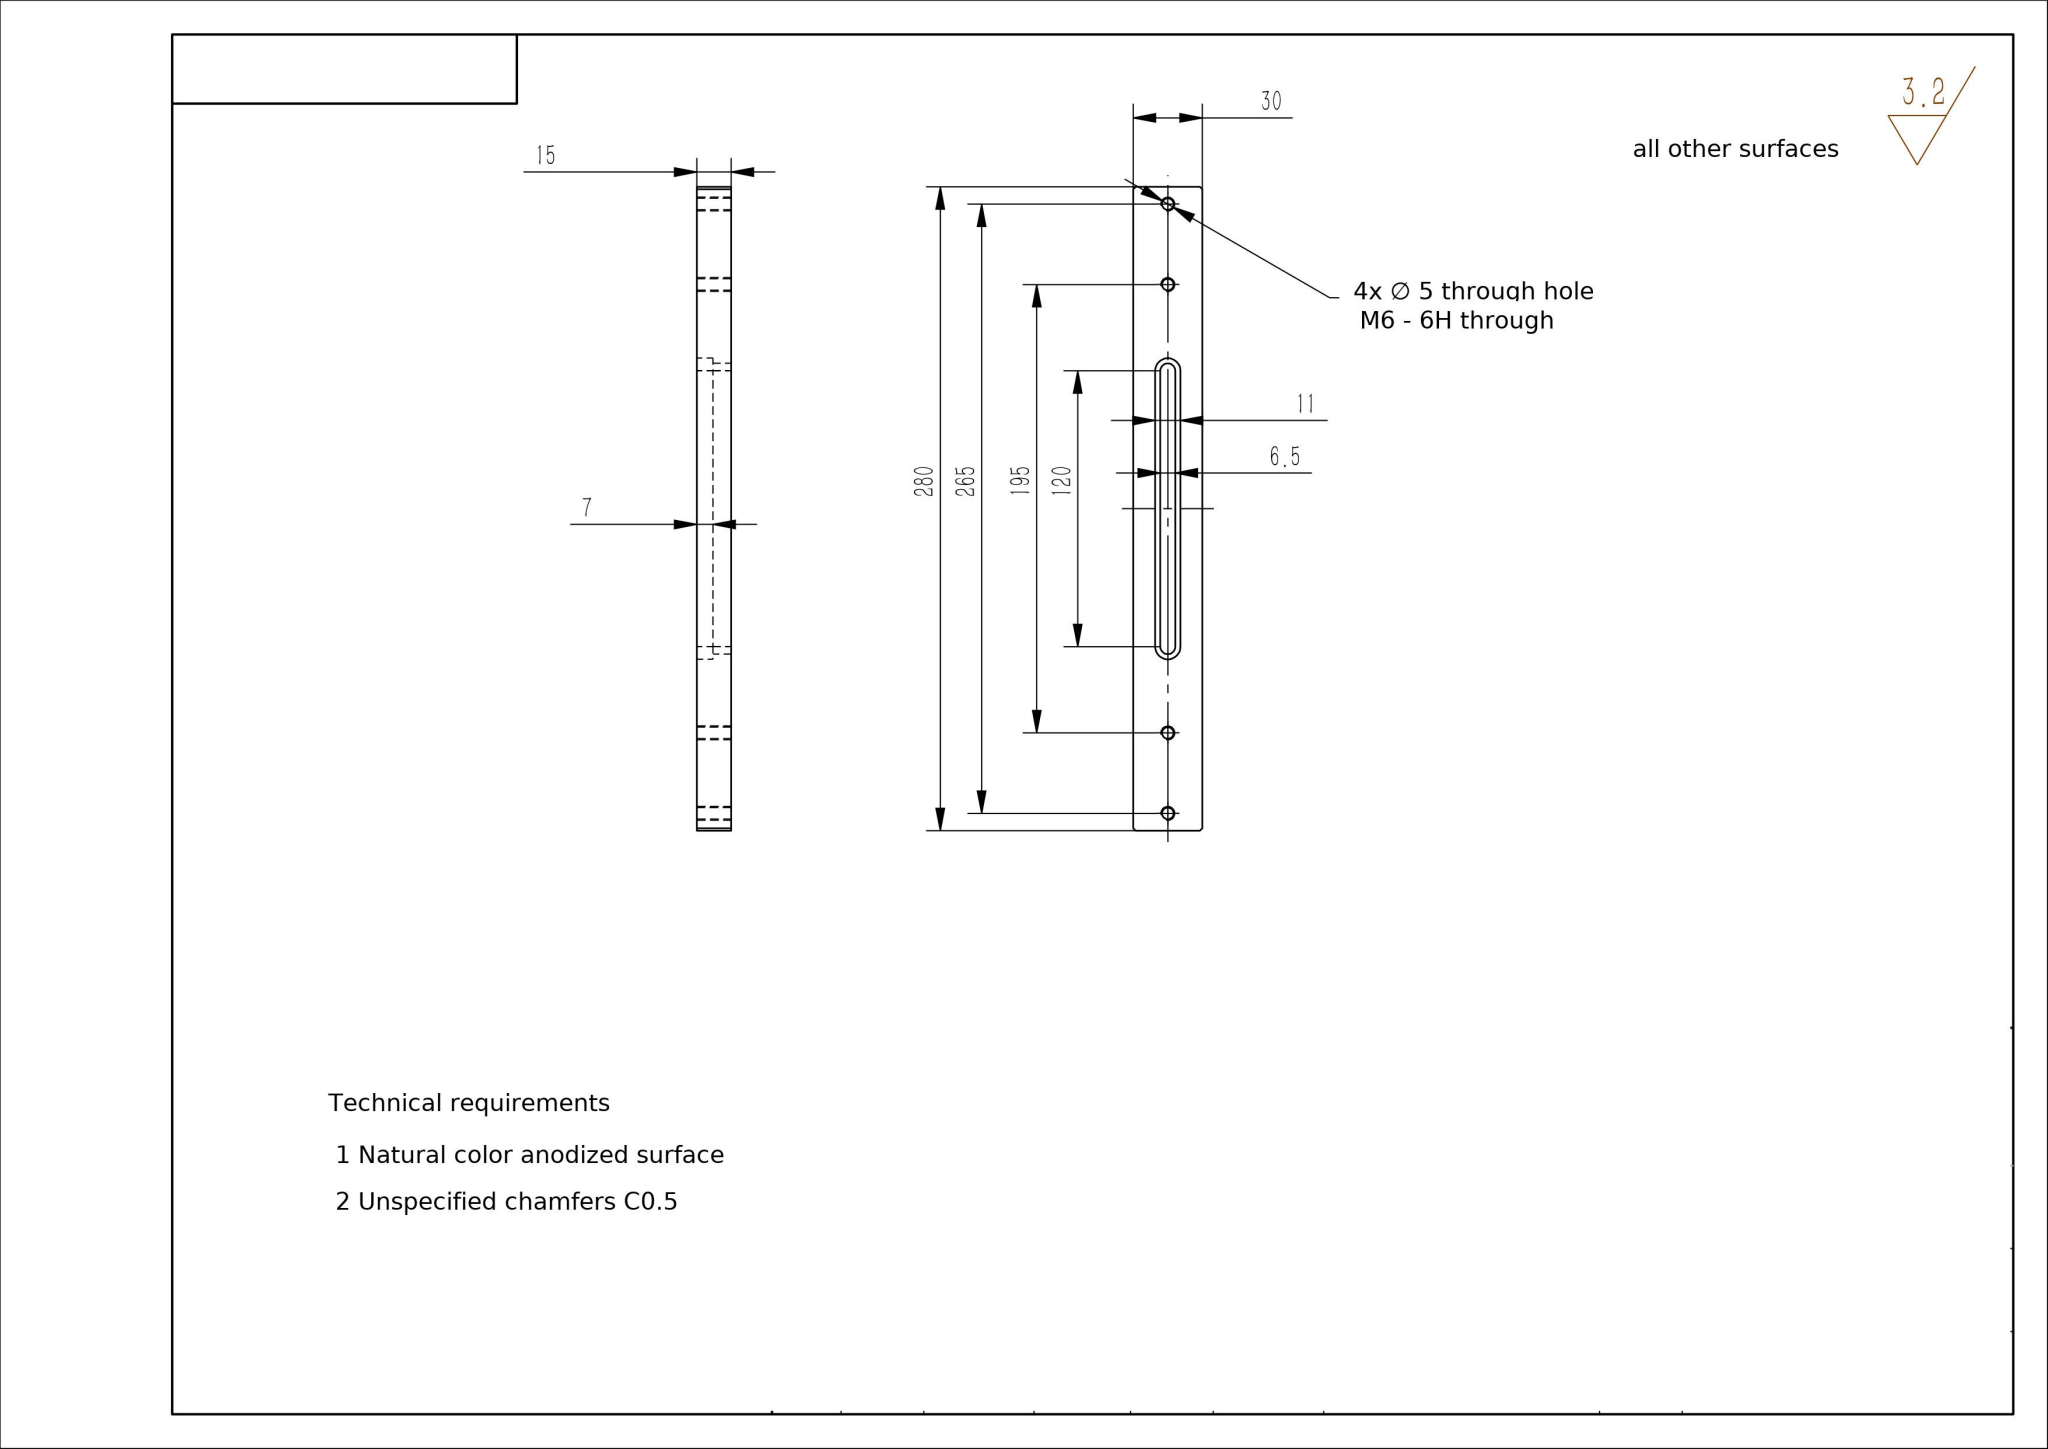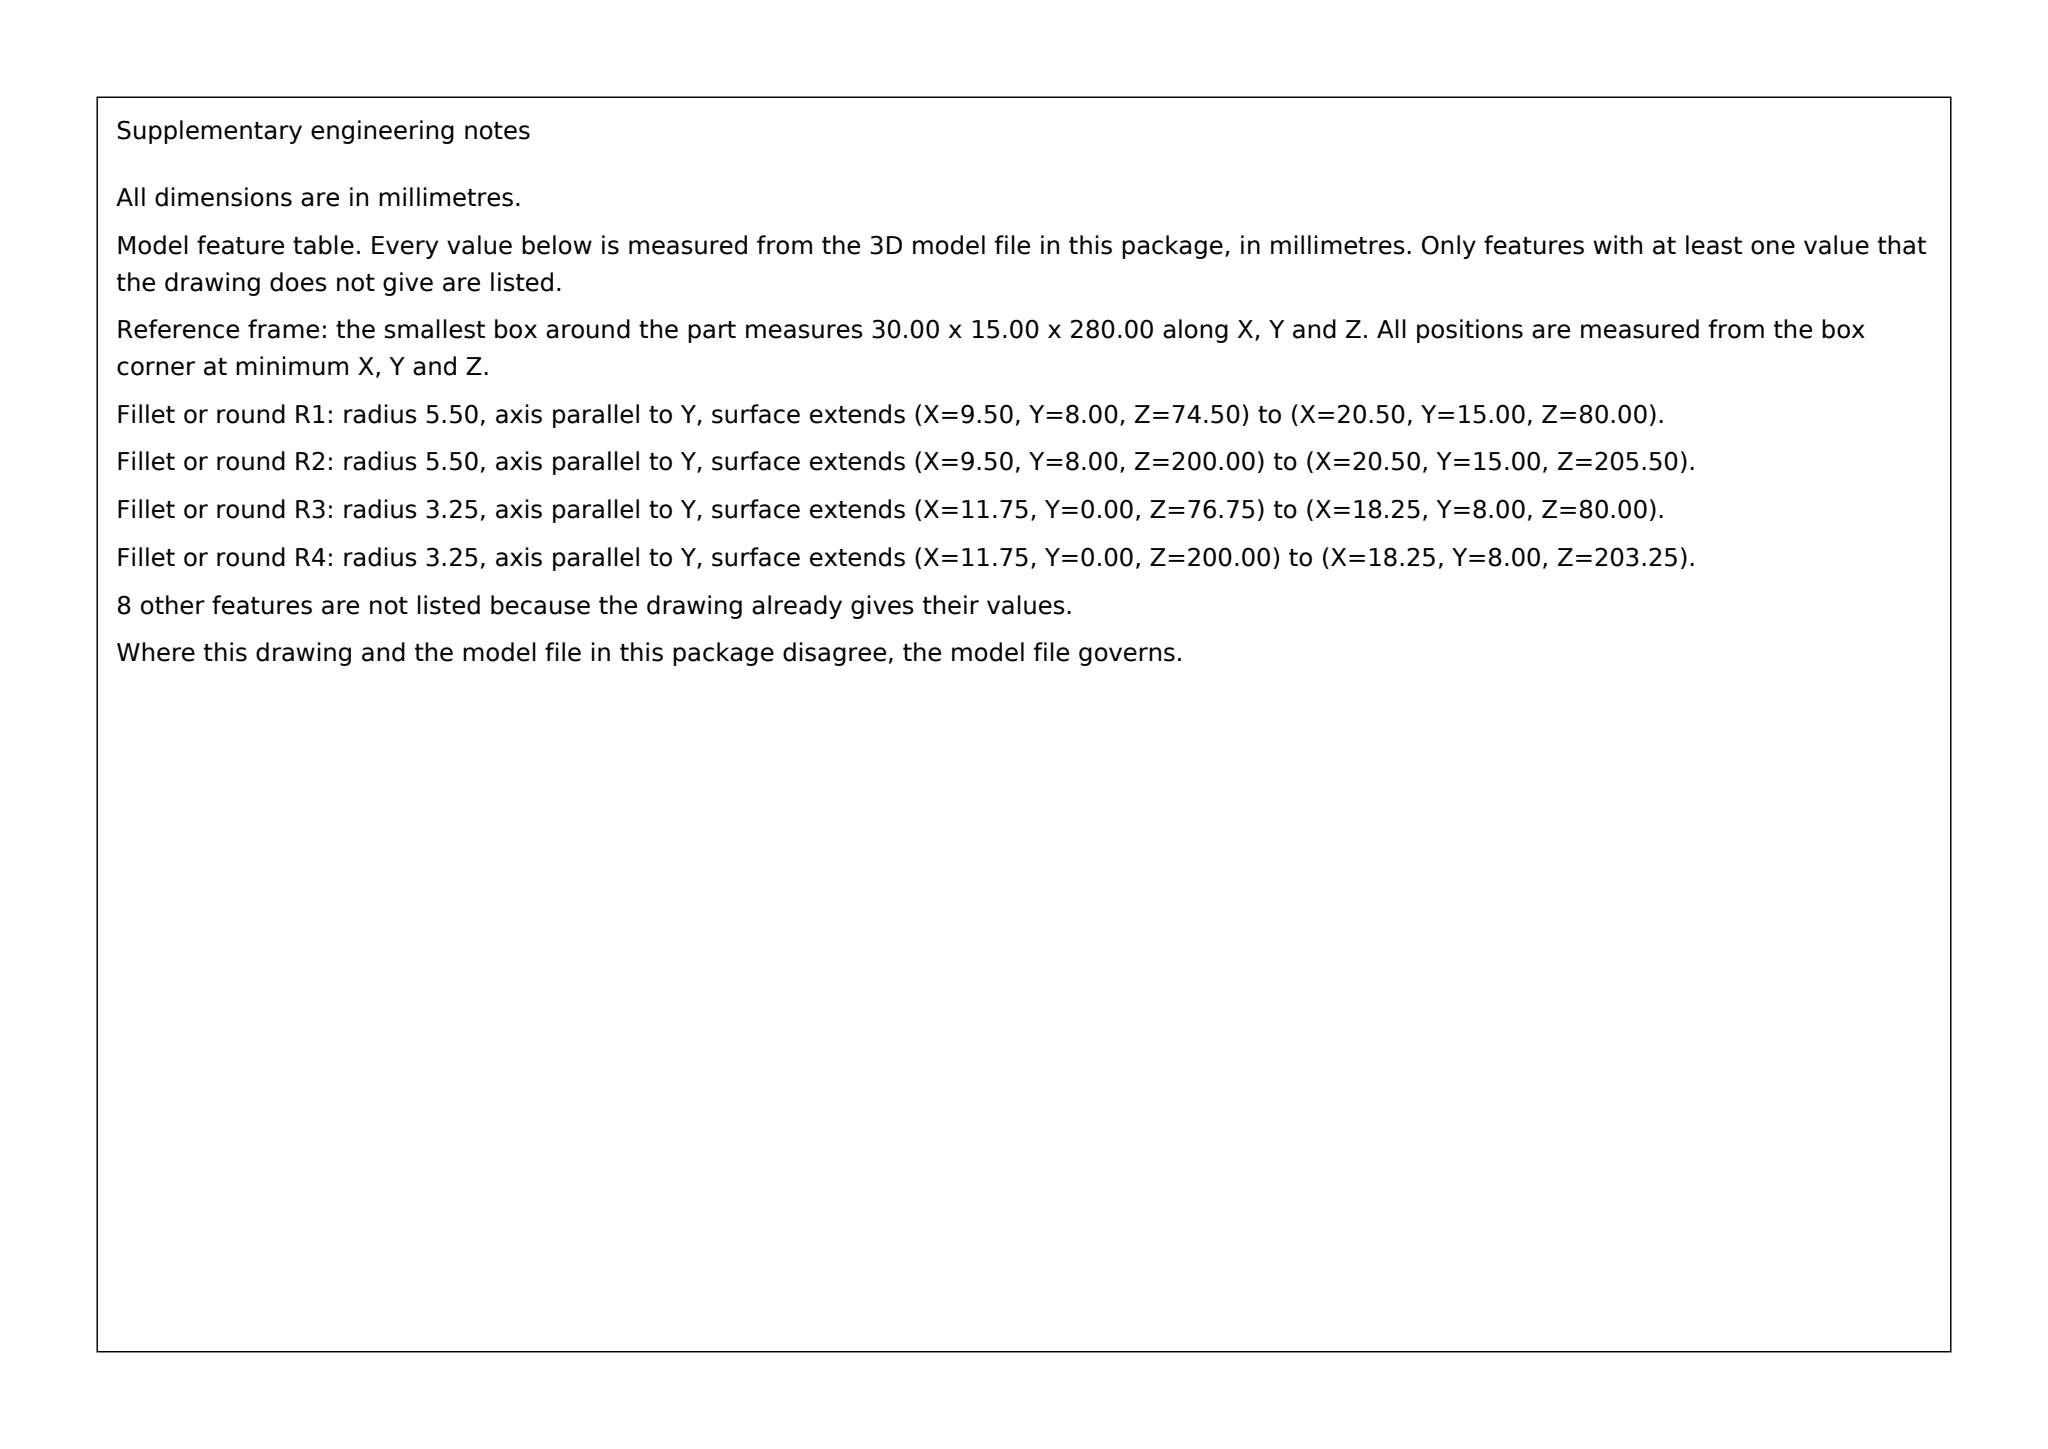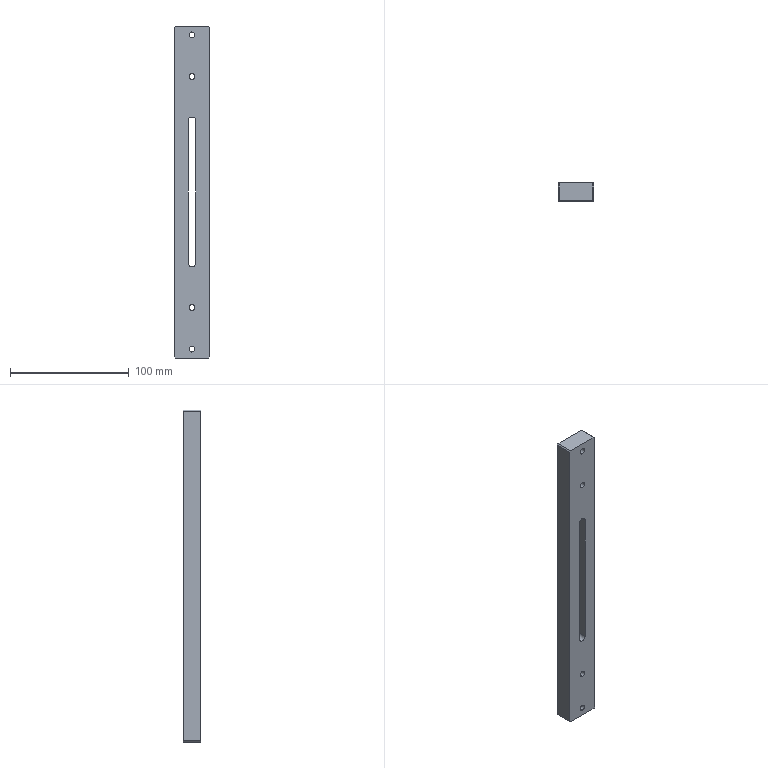Part | SolidWorks | mm | 1 solid | 29 faces | box 30 x 15 x 280 mm | volume 108381 mm3 | plane 15 | cylinder 14 | commonest cylinder face diameters 5 x8 6.5 x3 11 x3
build123d program:
from build123d import *

# Parameters (mm, degrees)
SKETCH1_W           = 30
SKETCH1_H           = 280
BOSS_EXTRUDE1_DEPTH = 15
M6_TAPPED_HOLE1_D   = 5
CHAMFER1_SIZE       = 1
CUT_EXTRUDE1_DEPTH  = 7
CUT_EXTRUDE2_DEPTH  = 142.028


with BuildPart() as part:
    # Sketch1 → Boss-Extrude1 (new body)
    with BuildSketch(Plane(origin=(0, 0, 0), x_dir=(1, 0, 0), z_dir=(0, 1, 0))):
        Rectangle(SKETCH1_W, SKETCH1_H)
    extrude(amount=BOSS_EXTRUDE1_DEPTH)

    # M6 Tapped Hole1 (through all)
    with Locations(Plane(origin=(0, 15, 0), x_dir=(1, 0, 0), z_dir=(0, 1, 0))):
        with Locations((0, -132.5), (0, -97.5), (0, 97.5), (0, 132.5)):
            Hole(M6_TAPPED_HOLE1_D / 2)

    # Chamfer1
    chamfer1_edges = [part.edges().sort_by_distance(p)[0] for p in [
        (15, 7.5, 140),
        (-15, 7.5, 140),
        (-15, 7.5, -140),
        (15, 7.5, -140),
    ]]
    chamfer(chamfer1_edges, length=CHAMFER1_SIZE)

    # Sketch4 → Cut-Extrude1 (cut)
    with BuildSketch(Plane(origin=(0, 15, 0), x_dir=(1, 0, 0), z_dir=(0, 1, 0))):
        with BuildLine():
            Line((5.5, 60), (5.5, -60))
            ThreePointArc((5.5, -60), (0, -65.5), (-5.5, -60))
            Line((-5.5, -60), (-5.5, 60))
            ThreePointArc((-5.5, 60), (0, 65.5), (5.5, 60))
        make_face()
    extrude(amount=-CUT_EXTRUDE1_DEPTH, mode=Mode.SUBTRACT)

    # Sketch5 → Cut-Extrude2 (cut, through all)
    with BuildSketch(Plane(origin=(0, 8, 0), x_dir=(1, 0, 0), z_dir=(0, 1, 0))):
        with BuildLine():
            Line((3.25, 60), (3.25, -60))
            ThreePointArc((3.25, -60), (0, -63.25), (-3.25, -60))
            Line((-3.25, -60), (-3.25, 60))
            ThreePointArc((-3.25, 60), (0, 63.25), (3.25, 60))
        make_face()
    extrude(amount=-CUT_EXTRUDE2_DEPTH, mode=Mode.SUBTRACT)


solid = part.part